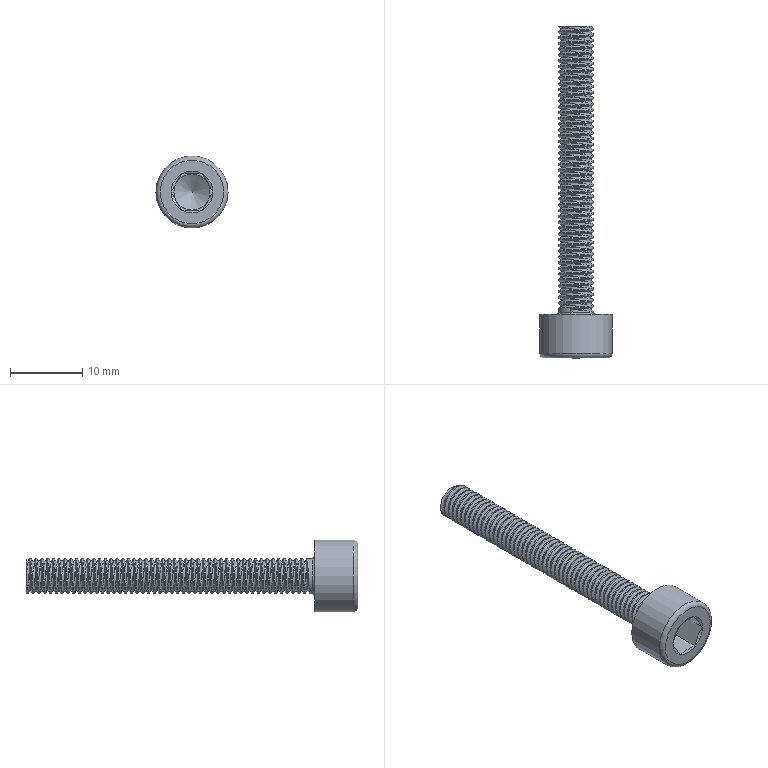Component | NX | M5_HEX_BOLT_2 | 1 solid | 30 faces | volume 1001 mm3 | plane 16 | cone 7 | cylinder 3 | torus 2 | spline 2 | commonest cylinder face diameters 4.976 x1 10 x1 4.2 x1